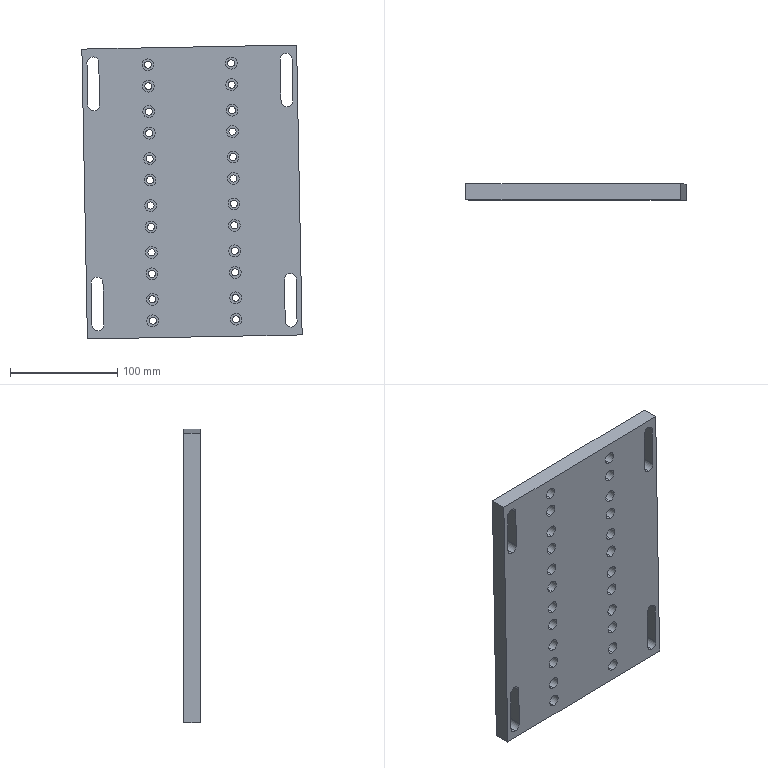Component | SolidWorks | 13TopPostMountingPlate-1 | 1 solid | 218 faces | box 205.11 x 15 x 273.76 mm | volume 745581 mm3 | cylinder 144 | plane 74 | commonest cylinder face diameters 11 x60 6.6 x48 10 x36 | material A3 Steel
build123d program:
from build123d import *

# Parameters (mm, degrees)
SKETCH1_W                                            = 270
SKETCH1_H                                            = 200
BOSS_EXTRUDE1_DEPTH                                  = 7.5
CUT_EXTRUDE1_DEPTH                                   = 169.671
HOLE_SIZE_ACCORDING_TO_HEXAGON_SOCKET_HE_D           = 6.6
HOLE_SIZE_ACCORDING_TO_HEXAGON_SOCKET_HE_CBORE_D     = 11
HOLE_SIZE_ACCORDING_TO_HEXAGON_SOCKET_HE_CBORE_DEPTH = 8.5
CUT_EXTRUDE2_DEPTH                                   = 2.5
LPATTERN1_COUNT                                      = 3
LPATTERN1_PITCH                                      = 43.7
MIRROR1_COPY_1_D                                     = 6.6
MIRROR1_COPY_1_CBORE_D                               = 11
MIRROR1_COPY_1_CBORE_DEPTH                           = 8.5
MIRROR1_COPY_2_D                                     = 6.6
MIRROR1_COPY_2_CBORE_D                               = 11
MIRROR1_COPY_2_CBORE_DEPTH                           = 8.5
MIRROR1_COPY_3_DEPTH                                 = 2.5
MIRROR1_COPY_4_DEPTH                                 = 2.5
MIRROR2_COPY_1_D                                     = 6.6
MIRROR2_COPY_1_CBORE_D                               = 11
MIRROR2_COPY_1_CBORE_DEPTH                           = 8.5
MIRROR2_COPY_2_D                                     = 6.6
MIRROR2_COPY_2_CBORE_D                               = 11
MIRROR2_COPY_2_CBORE_DEPTH                           = 8.5
MIRROR2_COPY_3_DEPTH                                 = 2.5
MIRROR2_COPY_4_DEPTH                                 = 2.5
MIRROR2_COPY_5_D                                     = 6.6
MIRROR2_COPY_5_CBORE_D                               = 11
MIRROR2_COPY_5_CBORE_DEPTH                           = 8.5
MIRROR2_COPY_6_DEPTH                                 = 2.5
MIRROR2_COPY_7_D                                     = 6.6
MIRROR2_COPY_7_CBORE_D                               = 11
MIRROR2_COPY_7_CBORE_DEPTH                           = 8.5
MIRROR2_COPY_8_D                                     = 6.6
MIRROR2_COPY_8_CBORE_D                               = 11
MIRROR2_COPY_8_CBORE_DEPTH                           = 8.5
MIRROR2_COPY_9_DEPTH                                 = 2.5
MIRROR2_COPY_10_DEPTH                                = 2.5


with BuildPart() as part:
    # Sketch1 → Boss-Extrude1 (new, symmetric)
    with BuildSketch(Plane.XY):
        Rectangle(SKETCH1_W, SKETCH1_H)
    extrude(amount=BOSS_EXTRUDE1_DEPTH, both=True)

    # Sketch2 → Cut-Extrude1 (cut, through all)
    with BuildSketch(Plane.XY.offset(7.5)):
        with BuildLine():
            Line((-122, 95.5), (-83, 95.5))
            ThreePointArc((-83, 95.5), (-77.5, 90), (-83, 84.5))
            Line((-83, 84.5), (-122, 84.5))
            ThreePointArc((-122, 84.5), (-127.5, 90), (-122, 95.5))
        make_face()
        with BuildLine():
            Line((122, 95.5), (83, 95.5))
            ThreePointArc((83, 95.5), (77.5, 90), (83, 84.5))
            Line((83, 84.5), (122, 84.5))
            ThreePointArc((122, 84.5), (127.5, 90), (122, 95.5))
        make_face()
        with BuildLine():
            Line((-122, -95.5), (-83, -95.5))
            ThreePointArc((-83, -95.5), (-77.5, -90), (-83, -84.5))
            Line((-83, -84.5), (-122, -84.5))
            ThreePointArc((-122, -84.5), (-127.5, -90), (-122, -95.5))
        make_face()
        with BuildLine():
            Line((122, -95.5), (83, -95.5))
            ThreePointArc((83, -95.5), (77.5, -90), (83, -84.5))
            Line((83, -84.5), (122, -84.5))
            ThreePointArc((122, -84.5), (127.5, -90), (122, -95.5))
        make_face()
    extrude(amount=-CUT_EXTRUDE1_DEPTH, mode=Mode.SUBTRACT)

    # Hole Size_According to_Hexagon Socket He (through all)
    with Locations(Plane(origin=(-31.85, 38.8, 7.5), x_dir=(1, 0, 0), z_dir=(0, 0, 1))):
        with Locations((0, 0), (20, 0)):
            hole_size_according_to_hexagon_socket_he = CounterBoreHole(HOLE_SIZE_ACCORDING_TO_HEXAGON_SOCKET_HE_D / 2, HOLE_SIZE_ACCORDING_TO_HEXAGON_SOCKET_HE_CBORE_D / 2, HOLE_SIZE_ACCORDING_TO_HEXAGON_SOCKET_HE_CBORE_DEPTH)

    # Sketch6 → Cut-Extrude2 (cut)
    with BuildSketch(Plane(origin=(0, 0, -7.5), x_dir=(-1, 0, 0), z_dir=(0, 0, -1))):
        with BuildLine():
            Line((8.6, 43.8), (35.1, 43.8))
            ThreePointArc((35.1, 43.8), (40.1, 38.8), (35.1, 33.8))
            Line((35.1, 33.8), (8.6, 33.8))
            ThreePointArc((8.6, 33.8), (3.6, 38.8), (8.6, 43.8))
        make_face()
    cut_extrude2 = extrude(amount=-CUT_EXTRUDE2_DEPTH, mode=Mode.SUBTRACT)

    # LPattern1: Hole Size_According to_Hexagon Socket He, Cut-Extrude2 ×3
    with Locations(*[(-i * LPATTERN1_PITCH, 0, 0) for i in range(1, LPATTERN1_COUNT)]):
        add(hole_size_according_to_hexagon_socket_he, mode=Mode.SUBTRACT)
        add(cut_extrude2, mode=Mode.SUBTRACT)

    # Mirror1: Hole Size_According to_Hexagon Socket He, Cut-Extrude2 across plane
    add(hole_size_according_to_hexagon_socket_he.mirror(Plane(origin=(0, 0, 0), x_dir=(0, 0, 1), z_dir=(1, 0, 0))), mode=Mode.SUBTRACT)
    add(cut_extrude2.mirror(Plane(origin=(0, 0, 0), x_dir=(0, 0, 1), z_dir=(1, 0, 0))), mode=Mode.SUBTRACT)

    # Mirror1 copy 1 (through all)
    with Locations(Plane(origin=(75.55, 38.8, 7.5), x_dir=(-1, 0, 0), z_dir=(0, 0, 1))):
        with Locations((0, 0), (20, 0)):
            CounterBoreHole(MIRROR1_COPY_1_D / 2, MIRROR1_COPY_1_CBORE_D / 2, MIRROR1_COPY_1_CBORE_DEPTH)

    # Mirror1 copy 2 (through all)
    with Locations(Plane(origin=(119.25, 38.8, 7.5), x_dir=(-1, 0, 0), z_dir=(0, 0, 1))):
        with Locations((0, 0), (20, 0)):
            CounterBoreHole(MIRROR1_COPY_2_D / 2, MIRROR1_COPY_2_CBORE_D / 2, MIRROR1_COPY_2_CBORE_DEPTH)

    # Mirror1 copy 3 sketch → Mirror1 copy 3 (cut)
    with BuildSketch(Plane(origin=(43.7, 0, -7.5), x_dir=(1, 0, 0), z_dir=(0, 0, -1))):
        with BuildLine():
            Line((8.6, -43.8), (35.1, -43.8))
            ThreePointArc((35.1, -43.8), (40.1, -38.8), (35.1, -33.8))
            Line((35.1, -33.8), (8.6, -33.8))
            ThreePointArc((8.6, -33.8), (3.6, -38.8), (8.6, -43.8))
        make_face()
    extrude(amount=-MIRROR1_COPY_3_DEPTH, mode=Mode.SUBTRACT)

    # Mirror1 copy 4 sketch → Mirror1 copy 4 (cut)
    with BuildSketch(Plane(origin=(87.4, 0, -7.5), x_dir=(1, 0, 0), z_dir=(0, 0, -1))):
        with BuildLine():
            Line((8.6, -43.8), (35.1, -43.8))
            ThreePointArc((35.1, -43.8), (40.1, -38.8), (35.1, -33.8))
            Line((35.1, -33.8), (8.6, -33.8))
            ThreePointArc((8.6, -33.8), (3.6, -38.8), (8.6, -43.8))
        make_face()
    extrude(amount=-MIRROR1_COPY_4_DEPTH, mode=Mode.SUBTRACT)

    # Mirror2: Hole Size_According to_Hexagon Socket He, Cut-Extrude2 across plane
    add(hole_size_according_to_hexagon_socket_he.mirror(Plane.ZX), mode=Mode.SUBTRACT)
    add(cut_extrude2.mirror(Plane.ZX), mode=Mode.SUBTRACT)

    # Mirror2 copy 1 (through all)
    with Locations(Plane(origin=(-75.55, -38.8, 7.5), x_dir=(1, 0, 0), z_dir=(0, 0, 1))):
        with Locations((0, 0), (20, 0)):
            CounterBoreHole(MIRROR2_COPY_1_D / 2, MIRROR2_COPY_1_CBORE_D / 2, MIRROR2_COPY_1_CBORE_DEPTH)

    # Mirror2 copy 2 (through all)
    with Locations(Plane(origin=(-119.25, -38.8, 7.5), x_dir=(1, 0, 0), z_dir=(0, 0, 1))):
        with Locations((0, 0), (20, 0)):
            CounterBoreHole(MIRROR2_COPY_2_D / 2, MIRROR2_COPY_2_CBORE_D / 2, MIRROR2_COPY_2_CBORE_DEPTH)

    # Mirror2 copy 3 sketch → Mirror2 copy 3 (cut)
    with BuildSketch(Plane(origin=(-43.7, 0, -7.5), x_dir=(-1, 0, 0), z_dir=(0, 0, -1))):
        with BuildLine():
            Line((8.6, -43.8), (35.1, -43.8))
            ThreePointArc((35.1, -43.8), (40.1, -38.8), (35.1, -33.8))
            Line((35.1, -33.8), (8.6, -33.8))
            ThreePointArc((8.6, -33.8), (3.6, -38.8), (8.6, -43.8))
        make_face()
    extrude(amount=-MIRROR2_COPY_3_DEPTH, mode=Mode.SUBTRACT)

    # Mirror2 copy 4 sketch → Mirror2 copy 4 (cut)
    with BuildSketch(Plane(origin=(-87.4, 0, -7.5), x_dir=(-1, 0, 0), z_dir=(0, 0, -1))):
        with BuildLine():
            Line((8.6, -43.8), (35.1, -43.8))
            ThreePointArc((35.1, -43.8), (40.1, -38.8), (35.1, -33.8))
            Line((35.1, -33.8), (8.6, -33.8))
            ThreePointArc((8.6, -33.8), (3.6, -38.8), (8.6, -43.8))
        make_face()
    extrude(amount=-MIRROR2_COPY_4_DEPTH, mode=Mode.SUBTRACT)

    # Mirror2 copy 5 (through all)
    with Locations(Plane(origin=(31.85, -38.8, 7.5), x_dir=(-1, 0, 0), z_dir=(0, 0, 1))):
        with Locations((0, 0), (20, 0)):
            CounterBoreHole(MIRROR2_COPY_5_D / 2, MIRROR2_COPY_5_CBORE_D / 2, MIRROR2_COPY_5_CBORE_DEPTH)

    # Mirror2 copy 6 sketch → Mirror2 copy 6 (cut)
    with BuildSketch(Plane(origin=(0, 0, -7.5), x_dir=(1, 0, 0), z_dir=(0, 0, -1))):
        with BuildLine():
            Line((8.6, 43.8), (35.1, 43.8))
            ThreePointArc((35.1, 43.8), (40.1, 38.8), (35.1, 33.8))
            Line((35.1, 33.8), (8.6, 33.8))
            ThreePointArc((8.6, 33.8), (3.6, 38.8), (8.6, 43.8))
        make_face()
    extrude(amount=-MIRROR2_COPY_6_DEPTH, mode=Mode.SUBTRACT)

    # Mirror2 copy 7 (through all)
    with Locations(Plane(origin=(75.55, -38.8, 7.5), x_dir=(-1, 0, 0), z_dir=(0, 0, 1))):
        with Locations((0, 0), (20, 0)):
            CounterBoreHole(MIRROR2_COPY_7_D / 2, MIRROR2_COPY_7_CBORE_D / 2, MIRROR2_COPY_7_CBORE_DEPTH)

    # Mirror2 copy 8 (through all)
    with Locations(Plane(origin=(119.25, -38.8, 7.5), x_dir=(-1, 0, 0), z_dir=(0, 0, 1))):
        with Locations((0, 0), (20, 0)):
            CounterBoreHole(MIRROR2_COPY_8_D / 2, MIRROR2_COPY_8_CBORE_D / 2, MIRROR2_COPY_8_CBORE_DEPTH)

    # Mirror2 copy 9 sketch → Mirror2 copy 9 (cut)
    with BuildSketch(Plane(origin=(43.7, 0, -7.5), x_dir=(1, 0, 0), z_dir=(0, 0, -1))):
        with BuildLine():
            Line((8.6, 43.8), (35.1, 43.8))
            ThreePointArc((35.1, 43.8), (40.1, 38.8), (35.1, 33.8))
            Line((35.1, 33.8), (8.6, 33.8))
            ThreePointArc((8.6, 33.8), (3.6, 38.8), (8.6, 43.8))
        make_face()
    extrude(amount=-MIRROR2_COPY_9_DEPTH, mode=Mode.SUBTRACT)

    # Mirror2 copy 10 sketch → Mirror2 copy 10 (cut)
    with BuildSketch(Plane(origin=(87.4, 0, -7.5), x_dir=(1, 0, 0), z_dir=(0, 0, -1))):
        with BuildLine():
            Line((8.6, 43.8), (35.1, 43.8))
            ThreePointArc((35.1, 43.8), (40.1, 38.8), (35.1, 33.8))
            Line((35.1, 33.8), (8.6, 33.8))
            ThreePointArc((8.6, 33.8), (3.6, 38.8), (8.6, 43.8))
        make_face()
    extrude(amount=-MIRROR2_COPY_10_DEPTH, mode=Mode.SUBTRACT)


solid = part.part

# Placed as in the assembly
solid = solid.moved(Location((1160.151, -1828.022, 2090.216), (90, 0, -88.909)))